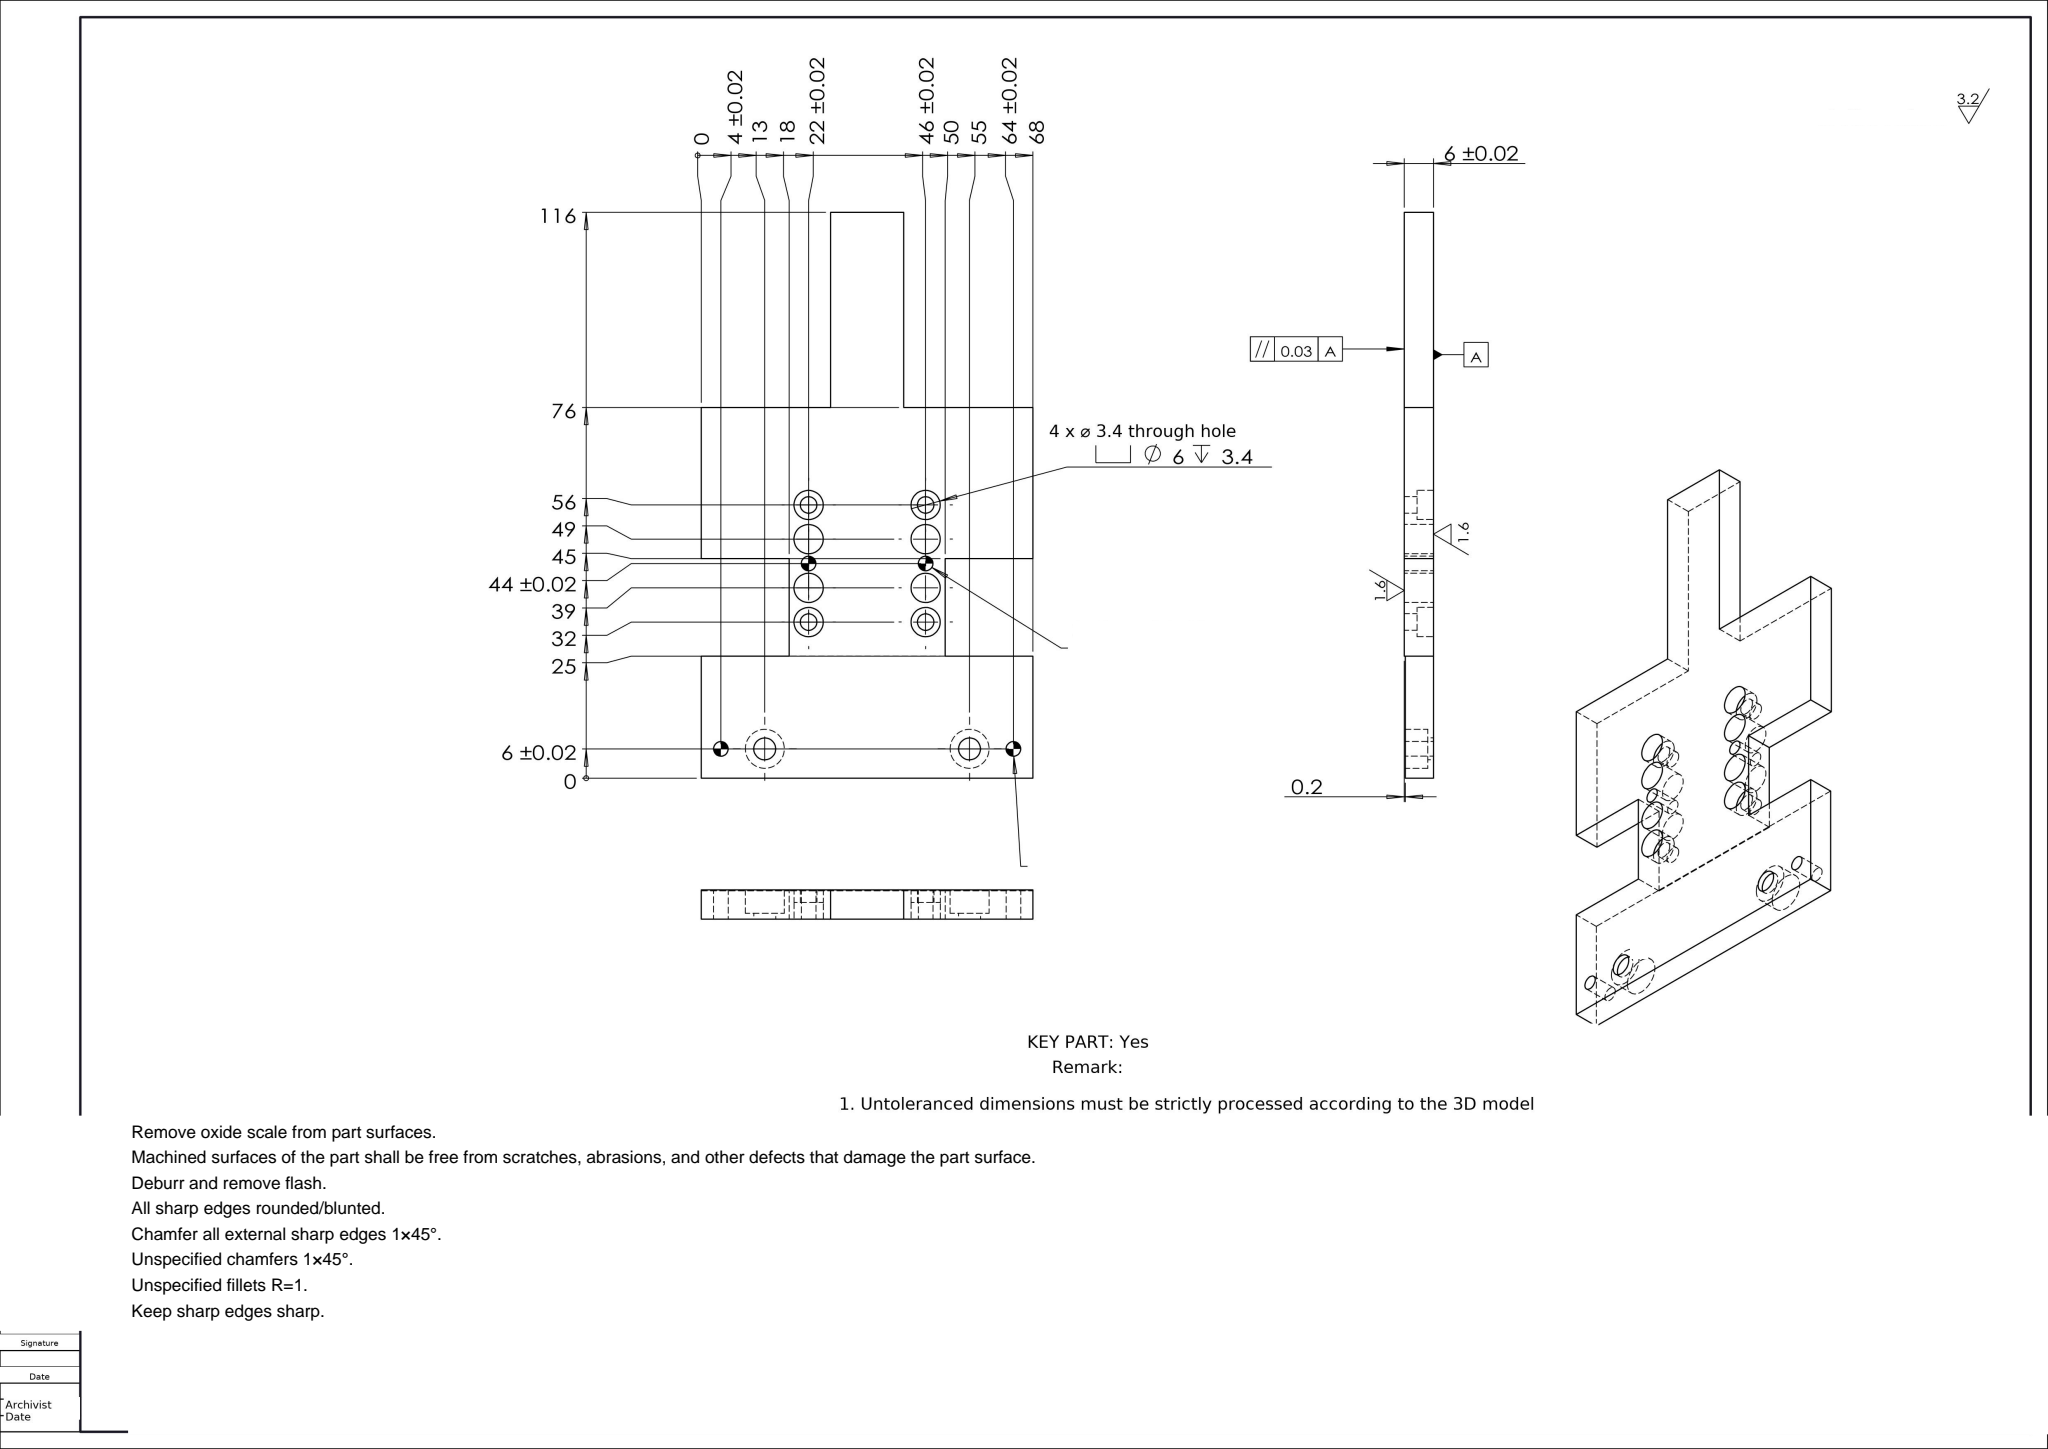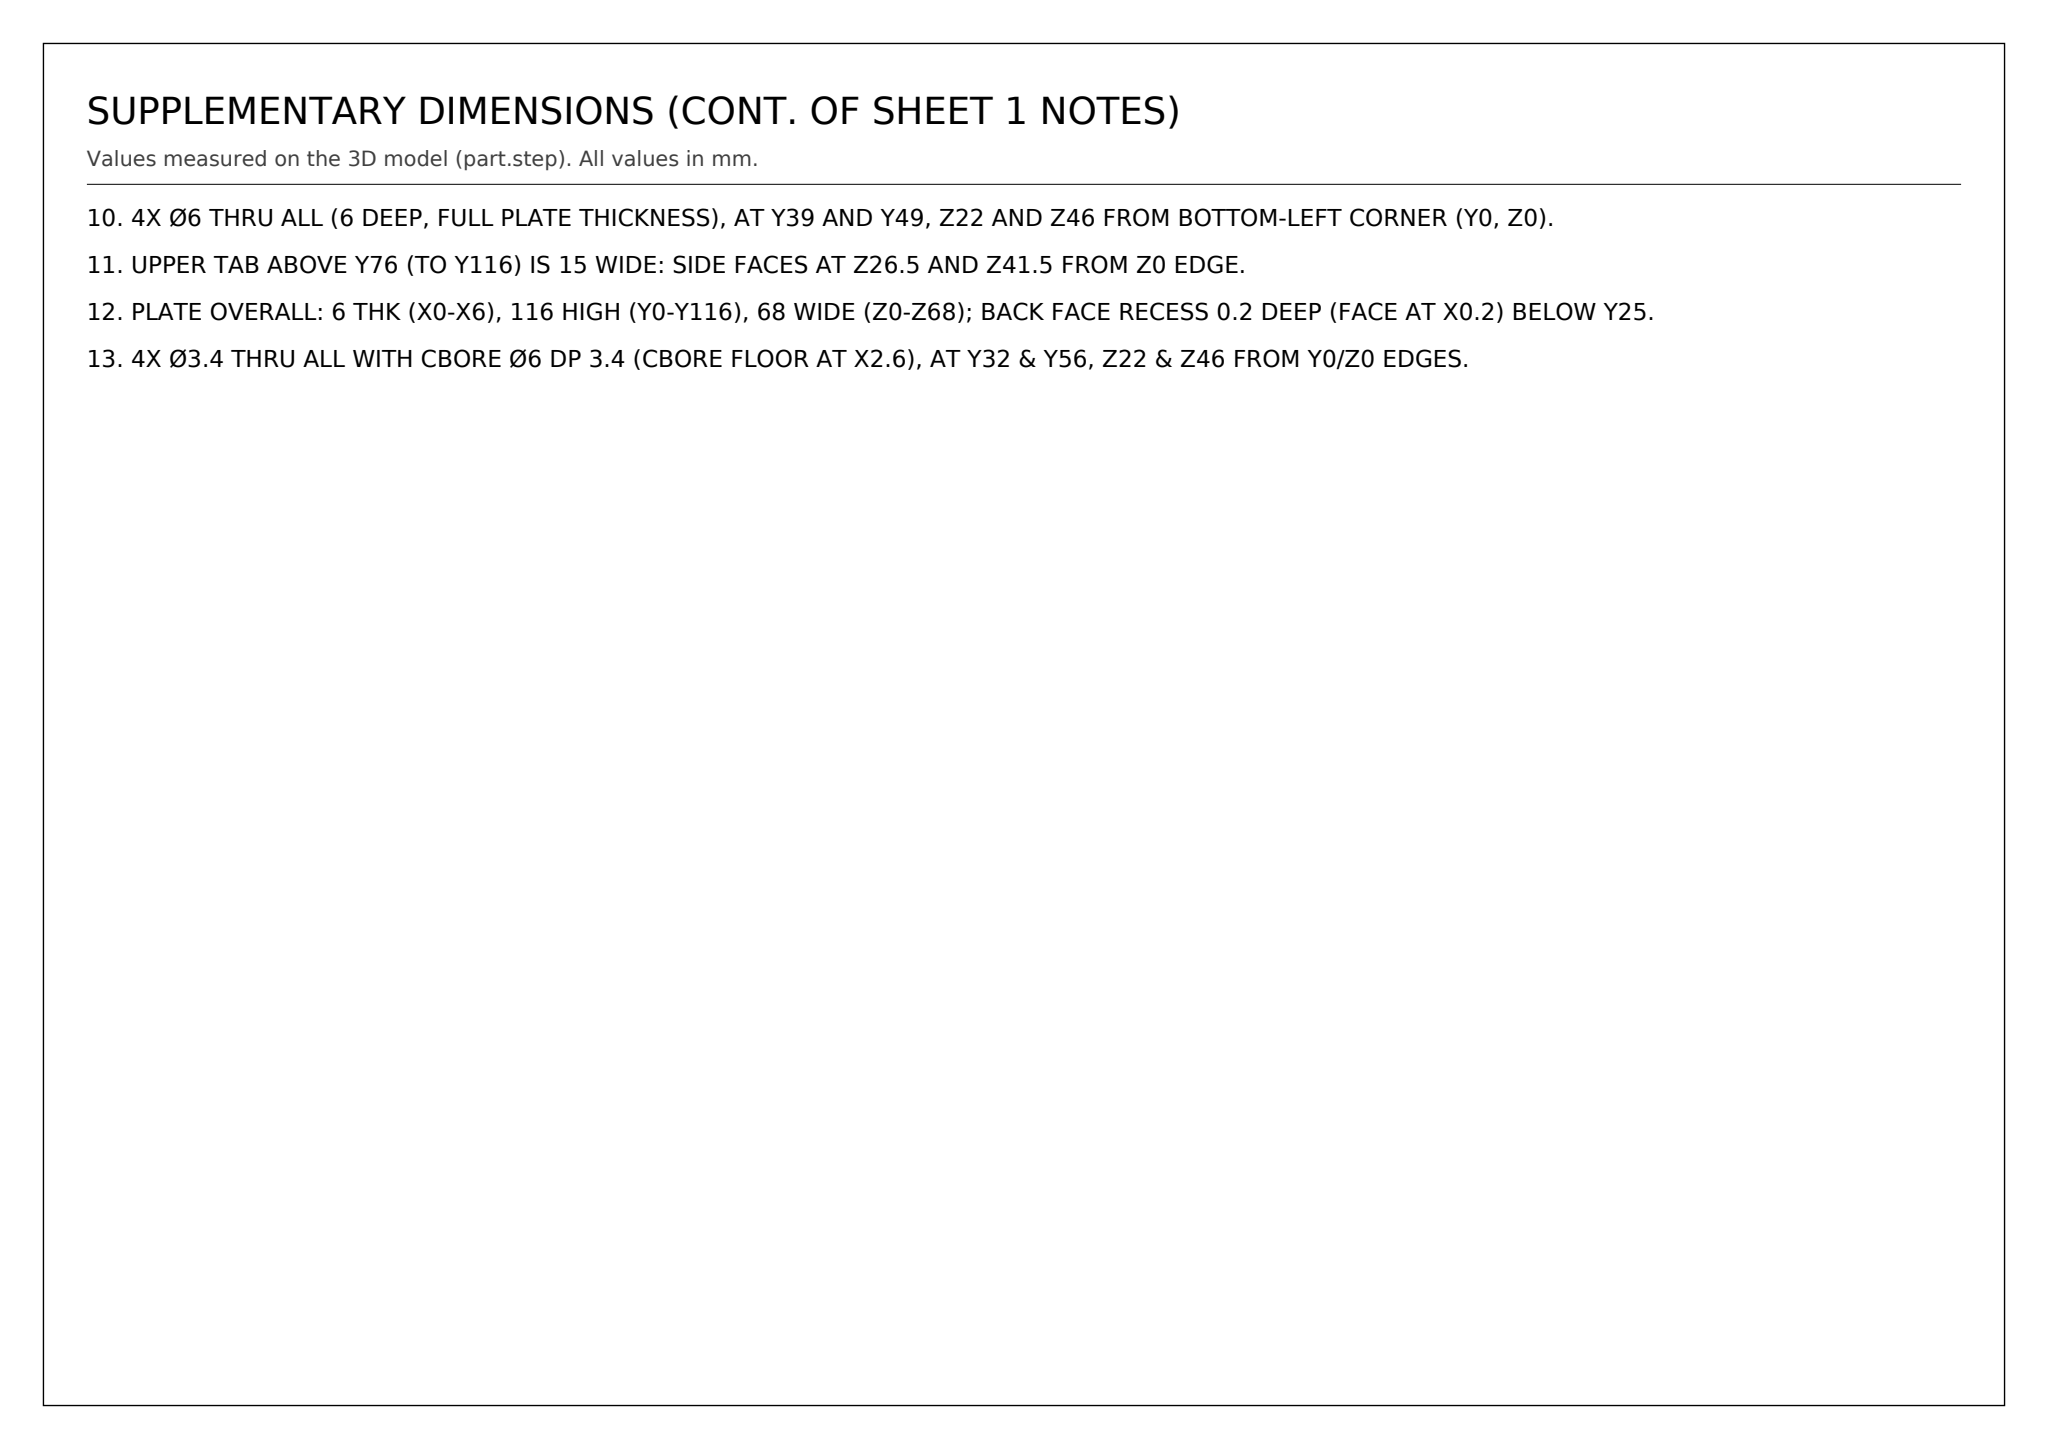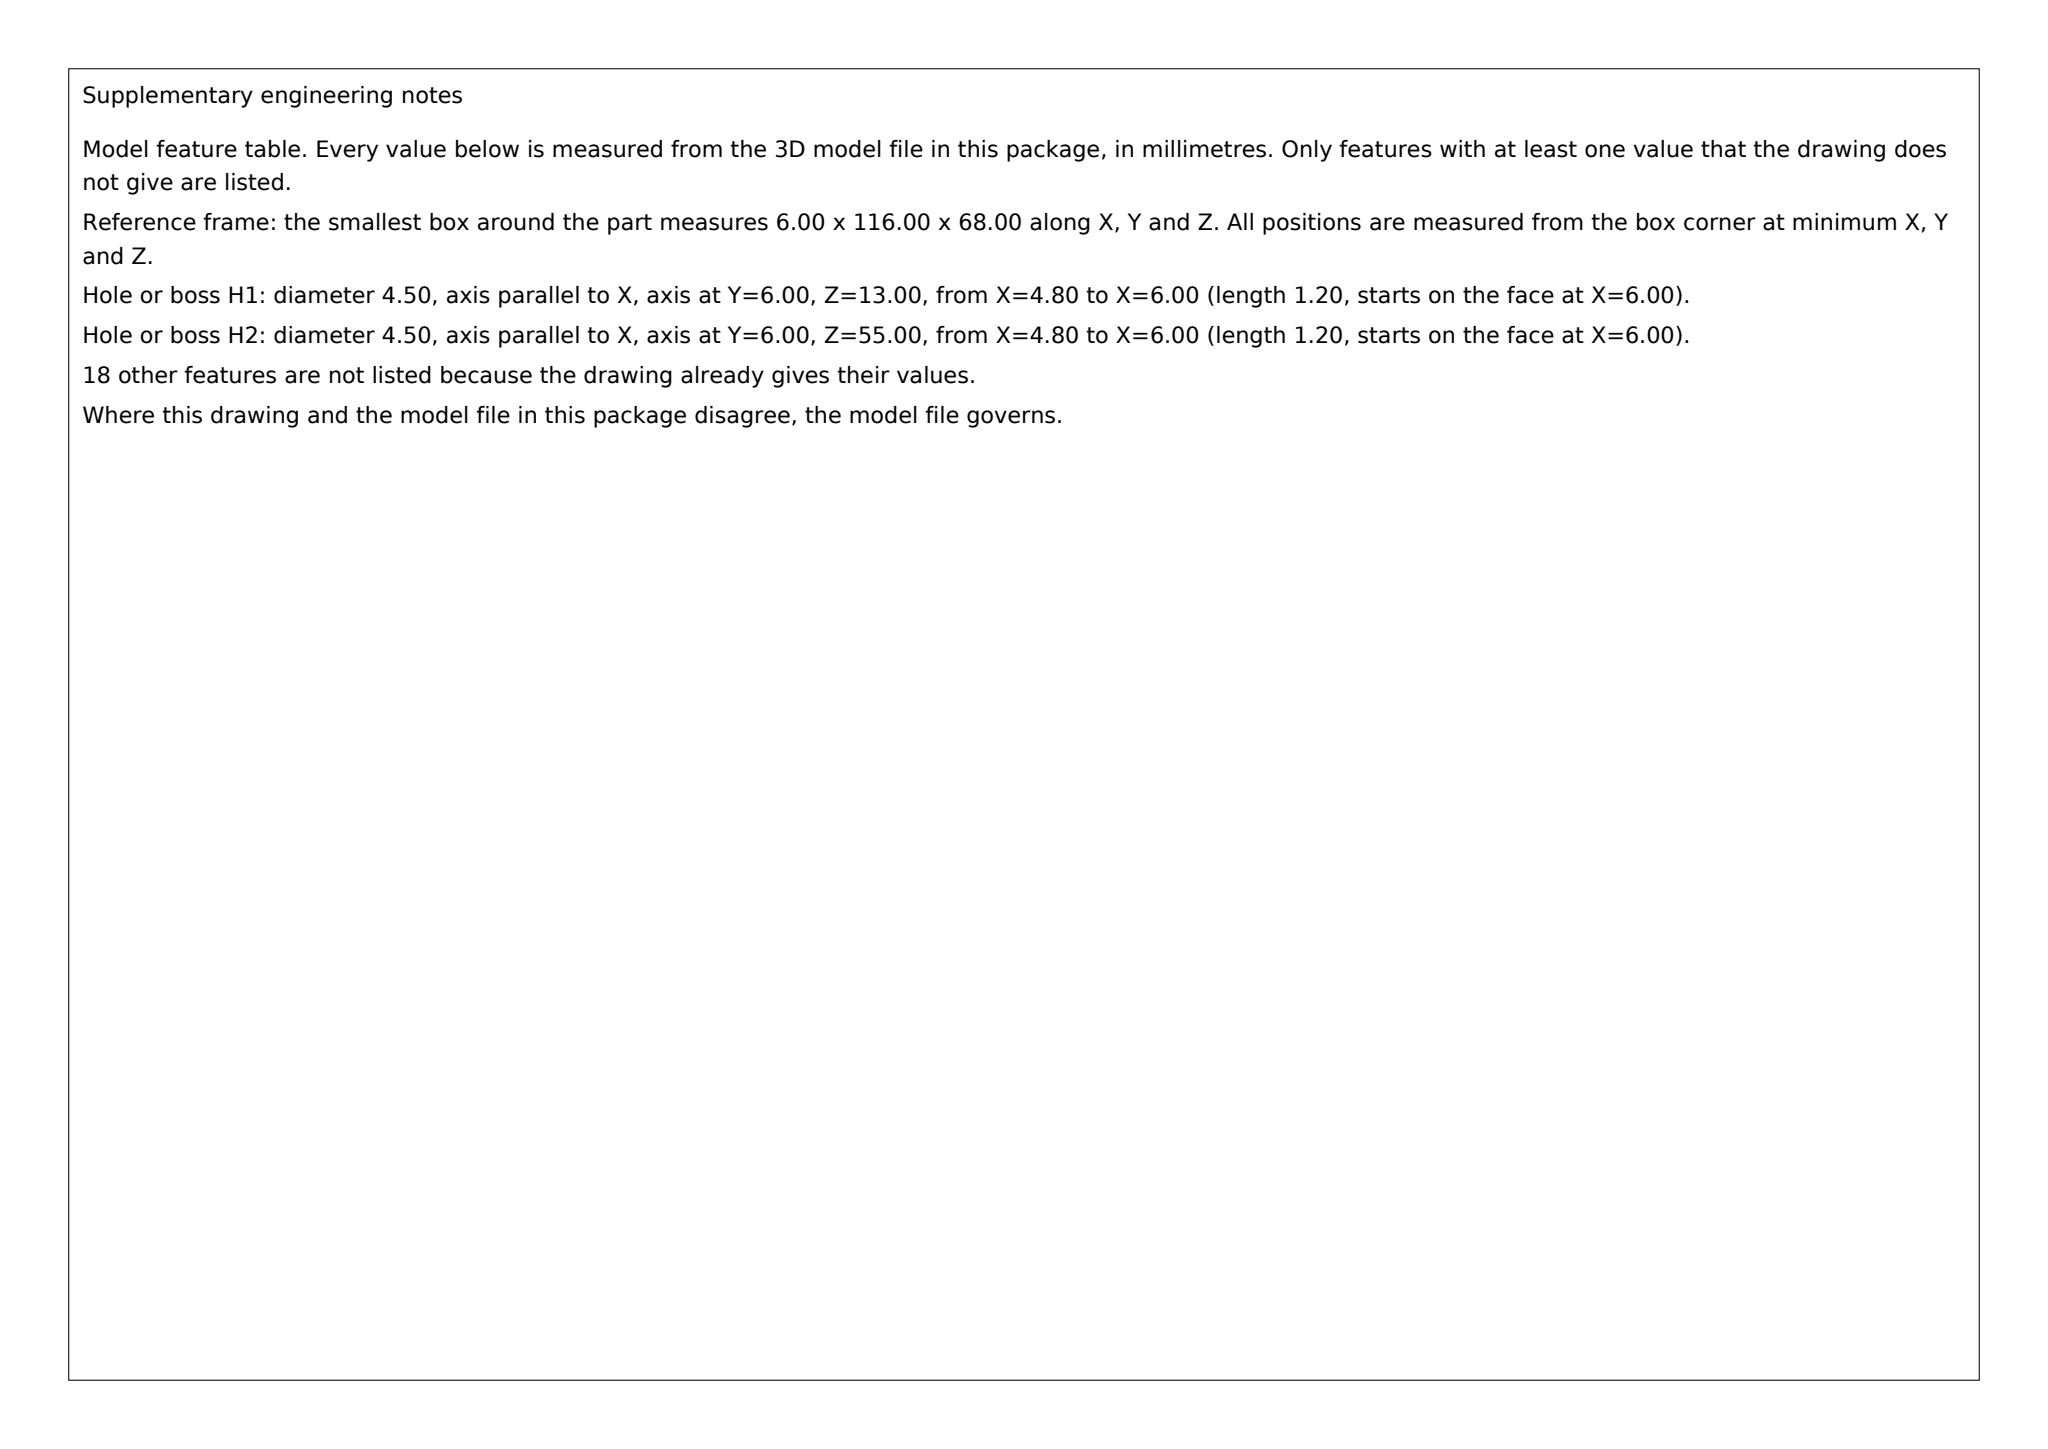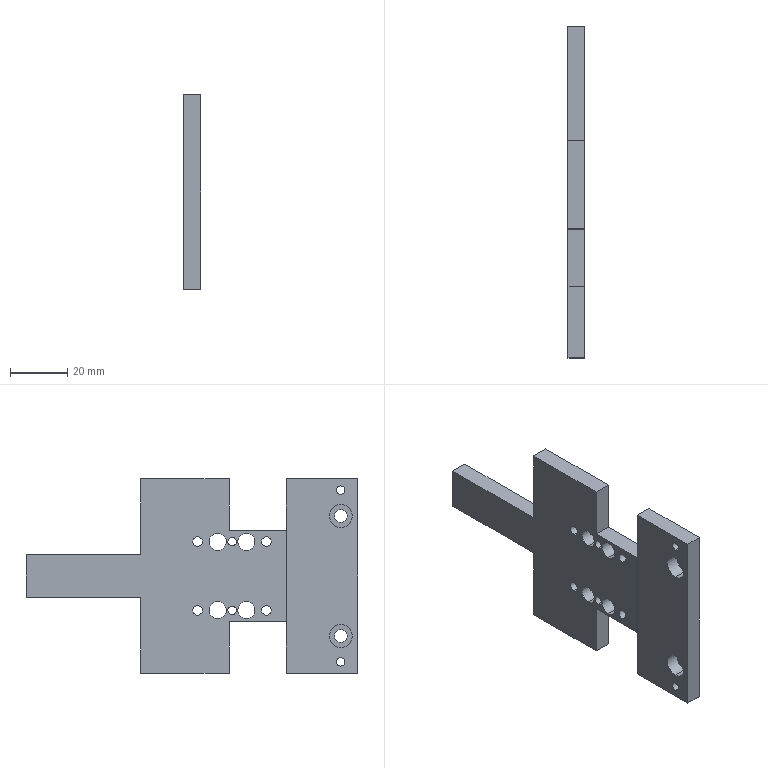Part | SolidWorks | mm | 1 solid | 66 faces | box 6 x 116 x 68 mm | volume 28123 mm3 | cylinder 40 | plane 26 | commonest cylinder face diameters 6 x16 3 x8 3.4 x8 8 x4 4.5 x4
Drawing notes:
BACK FACE RECESSED 0.2 DP BELOW Y25, FULL 68 WIDE | from the solid: axis_plane x=0.2 single face vs x=0 main face; recess bounded by y=25 planes (count 3) and z=0/z=68
2x Ø4.5 THRU, CBORE Ø8 DP 4.6 FROM RECESSED BACK FACE, AT Y6, Z13 & Z55 | from the solid: cylinders Ø4.5 x-axis at y=6, z=13 & 55 len 1.2 and Ø8 same pos len 4.6; 1.2+4.6=5.8=6.0-0.2
4X Ø6 THRU ALL, AT Y39 AND Y49, Z22 AND Z46 (FROM Y0 / Z0 EDGES) | from the solid: cylinders dia 6.0, axis x, at (y39,z22),(y39,z46),(y49,z22),(y49,z46), length 6.0 = full 6 mm plate thickness
UPPER TAB BETWEEN Y76 AND Y116 IS 15 WIDE: SIDE FACES AT Z26.5 AND Z41.5 FROM Z0 | from the solid: axis_planes normal z at offsets 26.5 and 41.5 (bbox z = 68)
2X Ø3 H7 (+0.010/0) THRU ALL, AT Y44, Z22 AND Z46 | from the solid: cylinders dia 3.0, axis x, at (y44,z22) and (y44,z46), length 6.0 = full thickness
2X Ø3 H7 (+0.010/0) THRU, 5.8 DEEP FROM 0.2 RECESSED BACK FACE, AT Y6, Z4 AND Z64 | from the solid: cylinders dia 3.0, axis x, at (y6,z4) and (y6,z64), length 5.8; axis_plane x = 0.2 (recessed back face)
4X Ø6 THRU ALL (6 DEEP, FULL 6 THK), AT Y39 & Y49 FROM Y0, Z22 & Z46 FROM Z0 | from the solid: cylinders: [6.0,"x",[null,39.0,22.0],6.0], [6.0,"x",[null,39.0,46.0],6.0], [6.0,"x",[null,49.0,22.0],6.0], [6.0,"x",[null,49.0,46.0],6.0]
UPPER TAB (Y76 TO Y116) IS 15 WIDE; SIDE FACES AT Z26.5 AND Z41.5 FROM Z0 | from the solid: axis_planes: ["z",26.5,1] and ["z",41.5,1] with ["y",76.0,2] / ["y",116.0,1]
OVERALL PLATE: 68 WIDE (Z0-Z68) X 116 HIGH (Y0-Y116) X 6 THK (X0-X6) | from the solid: bbox_xyz [6.0,116.0,68.0]; axis_planes x 0.0/6.0, y 0.0/116.0, z 0.0/68.0
4X Ø6 THRU ALL (6 DEEP, FULL PLATE THICKNESS), AT Y39 AND Y49, Z22 AND Z46 FROM BOTTOM-LEFT CORNER (Y0, Z0). | from the solid: cylinders: [6.0,'x',[null,39.0,22.0],6.0], [6.0,'x',[null,39.0,46.0],6.0], [6.0,'x',[null,49.0,22.0],6.0], [6.0,'x',[null,49.0,46.0],6.0]; bbox x=6.0
UPPER TAB ABOVE Y76 (TO Y116) IS 15 WIDE: SIDE FACES AT Z26.5 AND Z41.5 FROM Z0 EDGE. | from the solid: axis_planes: ['z',26.5,1], ['z',41.5,1] with ['y',76.0,2] and ['y',116.0,1]
PLATE OVERALL: 6 THK (X0-X6), 116 HIGH (Y0-Y116), 68 WIDE (Z0-Z68); BACK FACE RECESS 0.2 DEEP (FACE AT X0.2) BELOW Y25. | from the solid: bbox_xyz [6,116,68]; axis_planes x=0.0, x=0.2, y=25.0
4X Ø3.4 THRU ALL WITH CBORE Ø6 DP 3.4 (CBORE FLOOR AT X2.6), AT Y32 & Y56, Z22 & Z46 FROM Y0/Z0 EDGES. | from the solid: cylinders dia 3.4 len 2.6 at (32/56, 22/46) and dia 6.0 len 3.4 at same positions; axis_plane x=2.6
build123d program:
from build123d import *

# Parameters (mm, degrees)
SKETCH1_W                                         = 32
SKETCH1_H                                         = 38
BOSS_EXTRUDE1_DEPTH                               = 6
SKETCH2_W                                         = 68
SKETCH2_H                                         = 25
BOSS_EXTRUDE2_DEPTH                               = 5.8
SKETCH3_W                                         = 18
SKETCH3_H                                         = 18
BOSS_EXTRUDE3_DEPTH                               = 6
HOLE_WIZARD_K_D                                   = 6
SIZE_MM_DOWEL_PIN_HOLE1_D                         = 3
HOLE_SIZE_ACCORDING_TO_HEXAGON_SOCKET_D           = 3.4
HOLE_SIZE_ACCORDING_TO_HEXAGON_SOCKET_CBORE_D     = 6
HOLE_SIZE_ACCORDING_TO_HEXAGON_SOCKET_CBORE_DEPTH = 3.4
HOLE_SIZE_ACCORDING_TO_HEXAGON_SO_2_D             = 4.5
HOLE_SIZE_ACCORDING_TO_HEXAGON_SO_2_CBORE_D       = 8
HOLE_SIZE_ACCORDING_TO_HEXAGON_SO_2_CBORE_DEPTH   = 4.6
SIZE_MM_DOWEL_PIN_HOLE2_D                         = 3
SKETCH15_W                                        = 68
SKETCH15_H                                        = 13
BOSS_EXTRUDE4_DEPTH                               = 6
SKETCH17_W                                        = 15
SKETCH17_H                                        = 40
BOSS_EXTRUDE6_DEPTH                               = 6


with BuildPart() as part:
    # Sketch1 → Boss-Extrude1 (new body)
    with BuildSketch(Plane(origin=(0, 0, 0), x_dir=(0, 0, -1), z_dir=(1, 0, 0))):
        Rectangle(SKETCH1_W, SKETCH1_H)
    extrude(amount=BOSS_EXTRUDE1_DEPTH)

    # Sketch2 → Boss-Extrude2 (add)
    with BuildSketch(Plane(origin=(6, 0, 0), x_dir=(0, 0, -1), z_dir=(1, 0, 0))):
        with Locations((0, -31.5)):
            Rectangle(SKETCH2_W, SKETCH2_H)
    extrude(amount=-BOSS_EXTRUDE2_DEPTH)

    # Sketch3 → Boss-Extrude3 (add)
    with BuildSketch(Plane.ZY):
        with Locations((25, 10)):
            Rectangle(SKETCH3_W, SKETCH3_H)
        with Locations((-25, 10)):
            Rectangle(SKETCH3_W, SKETCH3_H)
    extrude(amount=-BOSS_EXTRUDE3_DEPTH)

    # Hole Wizard K (through all)
    with Locations(Plane(origin=(6, 0, 0), x_dir=(0, 0, -1), z_dir=(1, 0, 0))):
        with Locations((-12, 5), (12, 5), (12, -5), (-12, -5)):
            Hole(HOLE_WIZARD_K_D / 2)

    # Size mm Dowel Pin Hole1 (through all)
    with Locations(Plane(origin=(6, 0, 0), x_dir=(0, 0, -1), z_dir=(1, 0, 0))):
        with Locations((-12, 0), (12, 0)):
            Hole(SIZE_MM_DOWEL_PIN_HOLE1_D / 2)

    # Hole Size _ according to_ Hexagon Socket (through all)
    with Locations(Plane(origin=(6, 0, 0), x_dir=(0, 0, -1), z_dir=(1, 0, 0))):
        with Locations((-12, 12), (12, 12), (-12, -12), (12, -12)):
            CounterBoreHole(HOLE_SIZE_ACCORDING_TO_HEXAGON_SOCKET_D / 2, HOLE_SIZE_ACCORDING_TO_HEXAGON_SOCKET_CBORE_D / 2, HOLE_SIZE_ACCORDING_TO_HEXAGON_SOCKET_CBORE_DEPTH)

    # Hole Size _ according to_ Hexagon So 2 (through all)
    with Locations(Plane.ZY.offset(-0.2)):
        with Locations((-21, -38), (21, -38)):
            CounterBoreHole(HOLE_SIZE_ACCORDING_TO_HEXAGON_SO_2_D / 2, HOLE_SIZE_ACCORDING_TO_HEXAGON_SO_2_CBORE_D / 2, HOLE_SIZE_ACCORDING_TO_HEXAGON_SO_2_CBORE_DEPTH)

    # Size mm Dowel Pin Hole2 (through all)
    with Locations(Plane.ZY.offset(-0.2)):
        with Locations((-30, -38), (30, -38)):
            Hole(SIZE_MM_DOWEL_PIN_HOLE2_D / 2)

    # Sketch15 → Boss-Extrude4 (add)
    with BuildSketch(Plane(origin=(6, 0, 0), x_dir=(0, 0, -1), z_dir=(1, 0, 0))):
        with Locations((0, 25.5)):
            Rectangle(SKETCH15_W, SKETCH15_H)
    extrude(amount=-BOSS_EXTRUDE4_DEPTH)

    # Sketch17 → Boss-Extrude6 (add)
    with BuildSketch(Plane(origin=(6, 0, 0), x_dir=(0, 0, -1), z_dir=(1, 0, 0))):
        with Locations((0, 52)):
            Rectangle(SKETCH17_W, SKETCH17_H)
    extrude(amount=-BOSS_EXTRUDE6_DEPTH)


solid = part.part